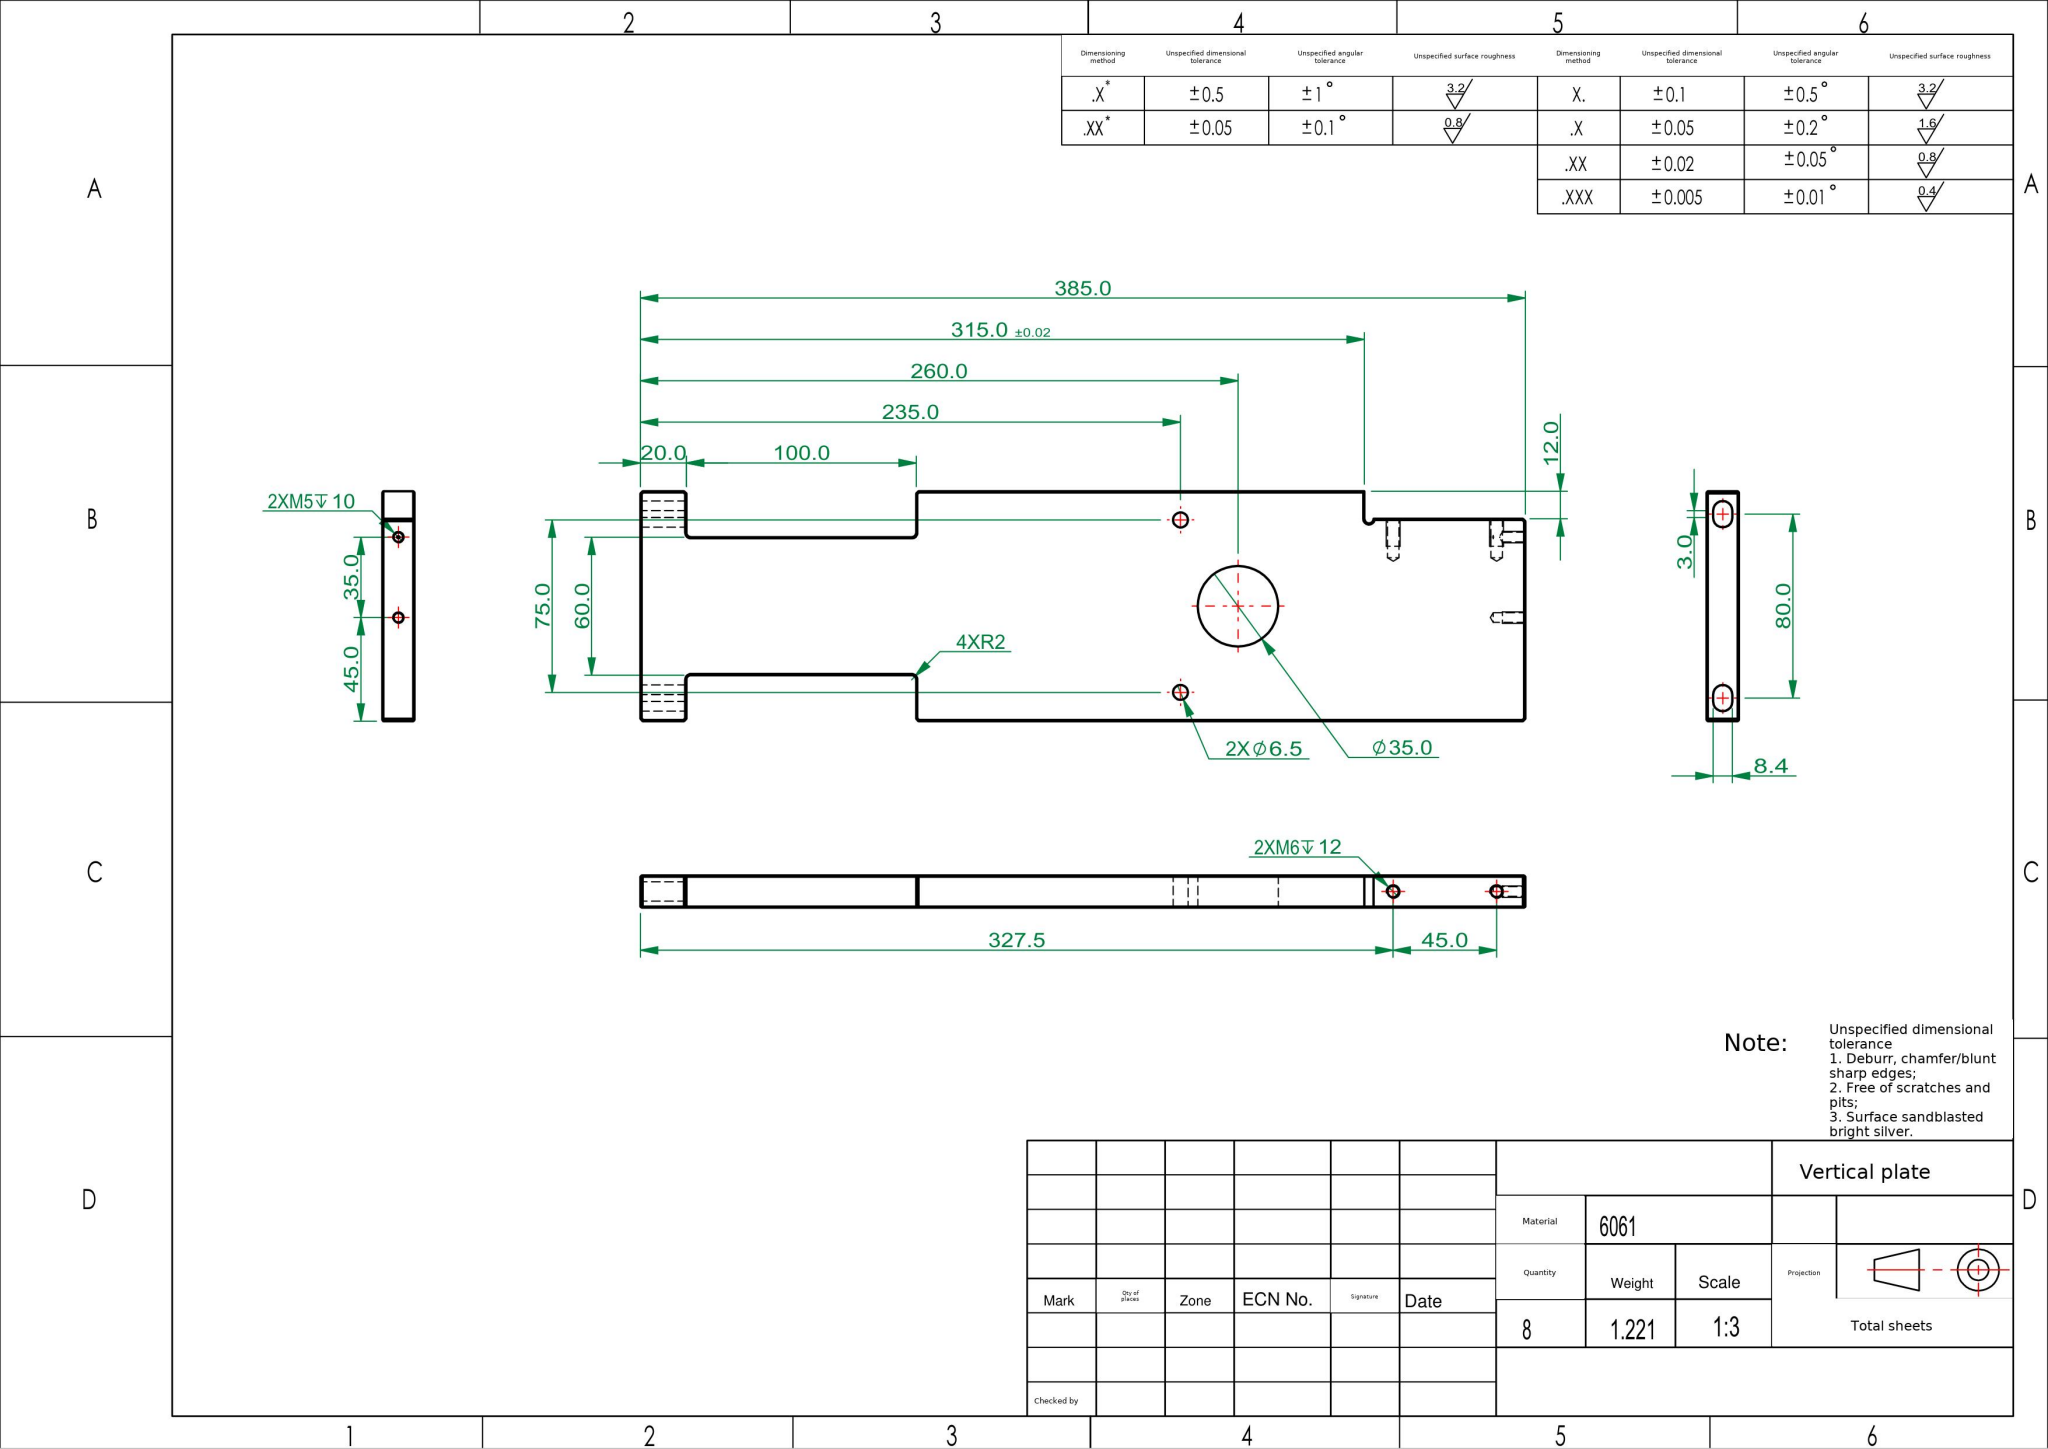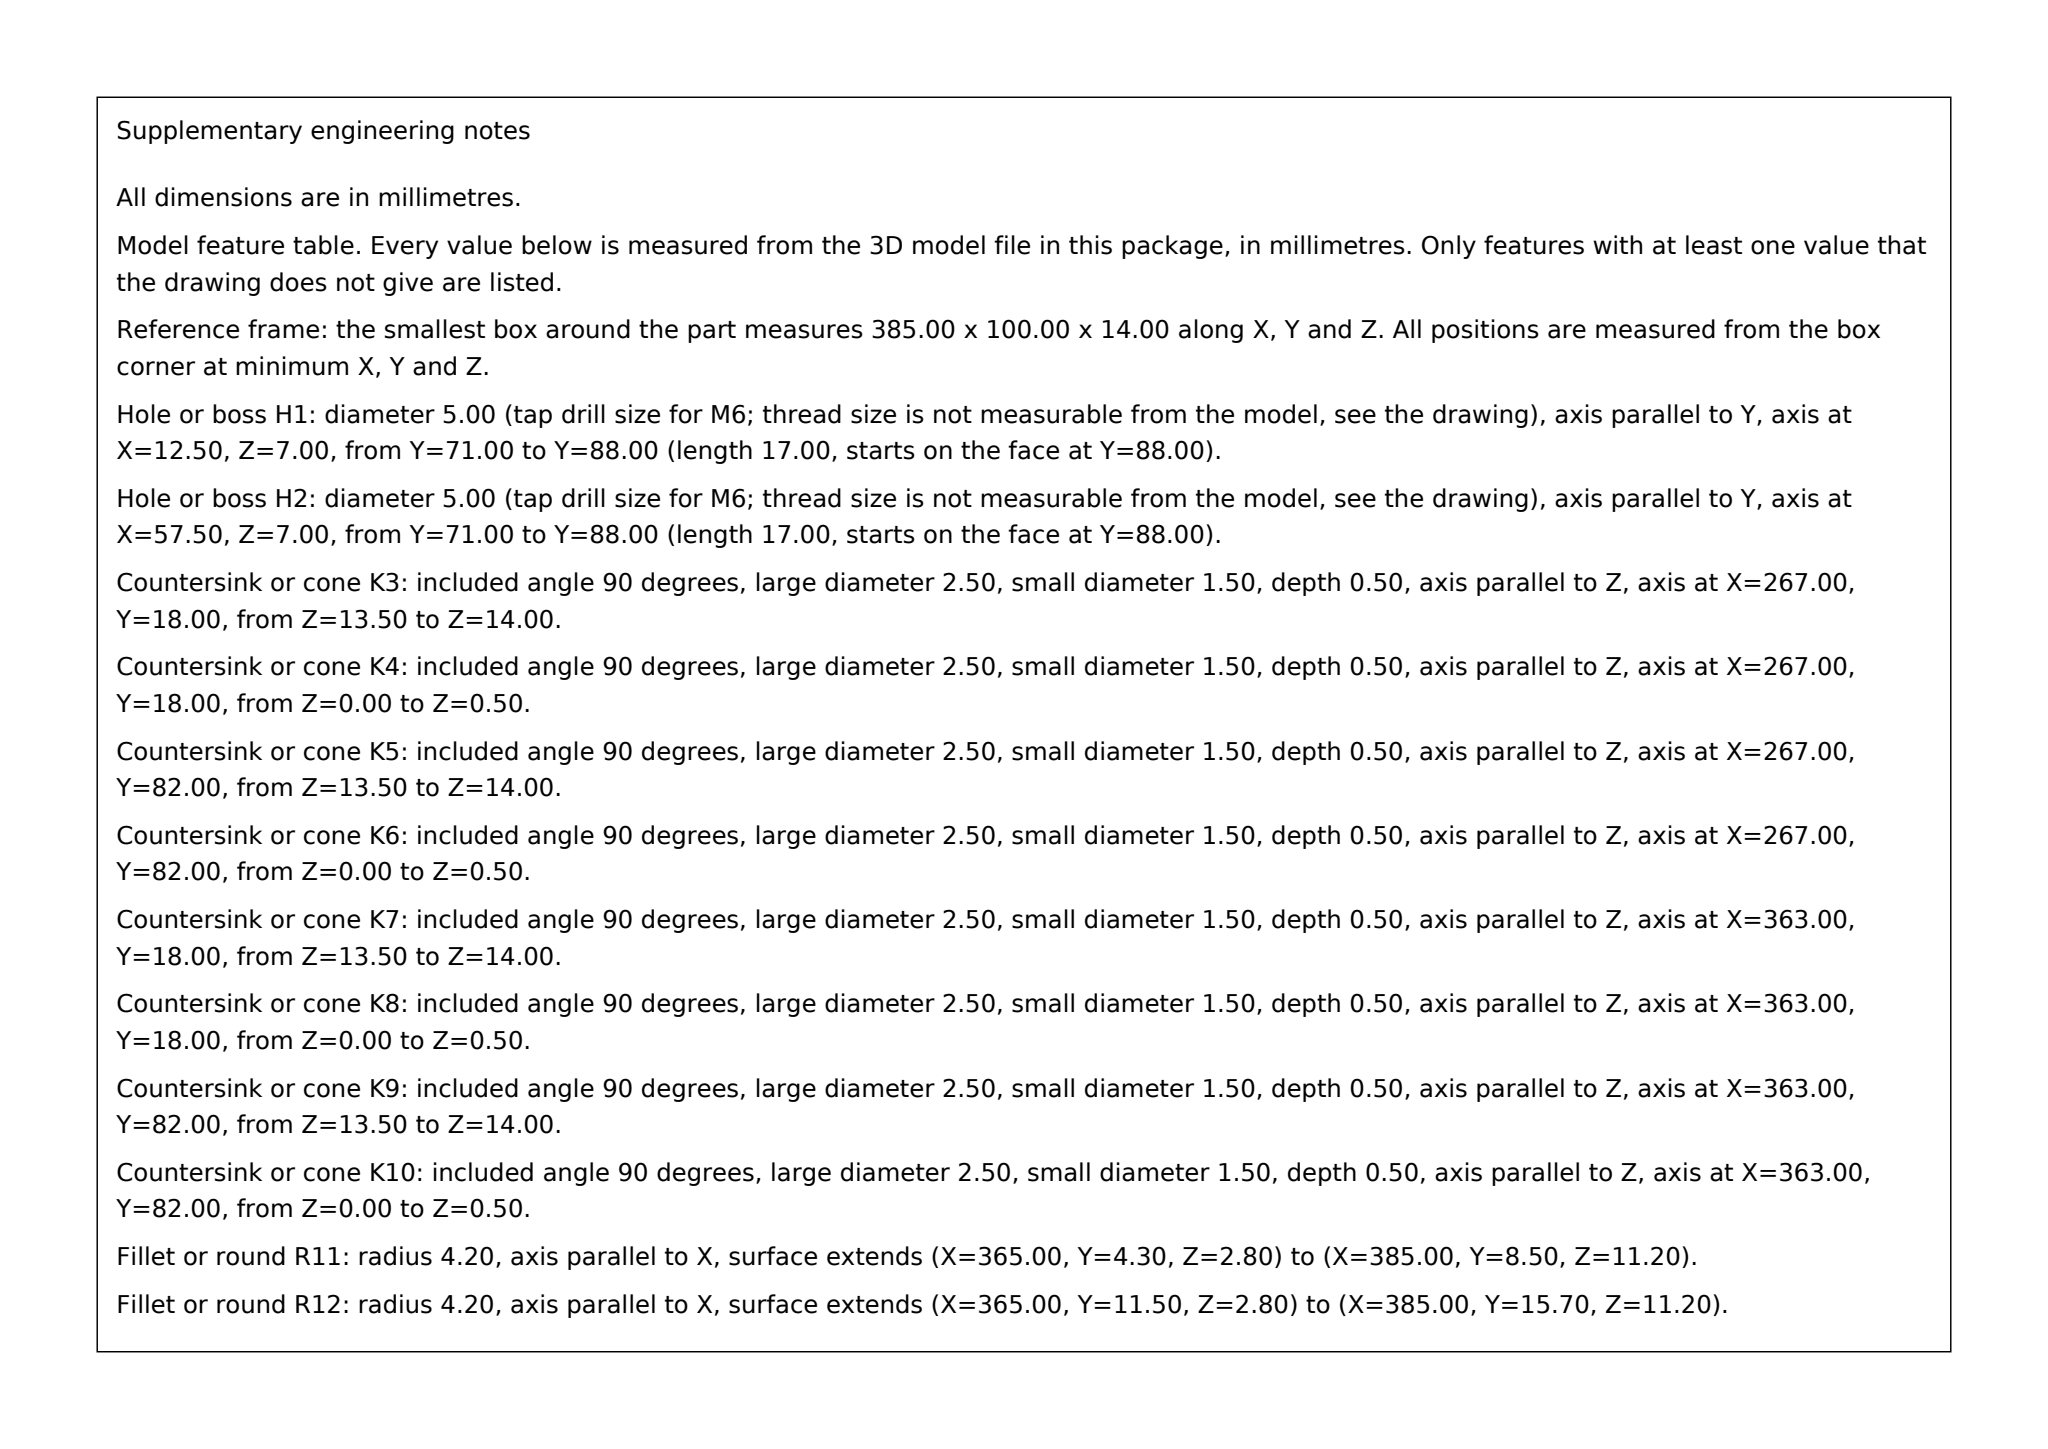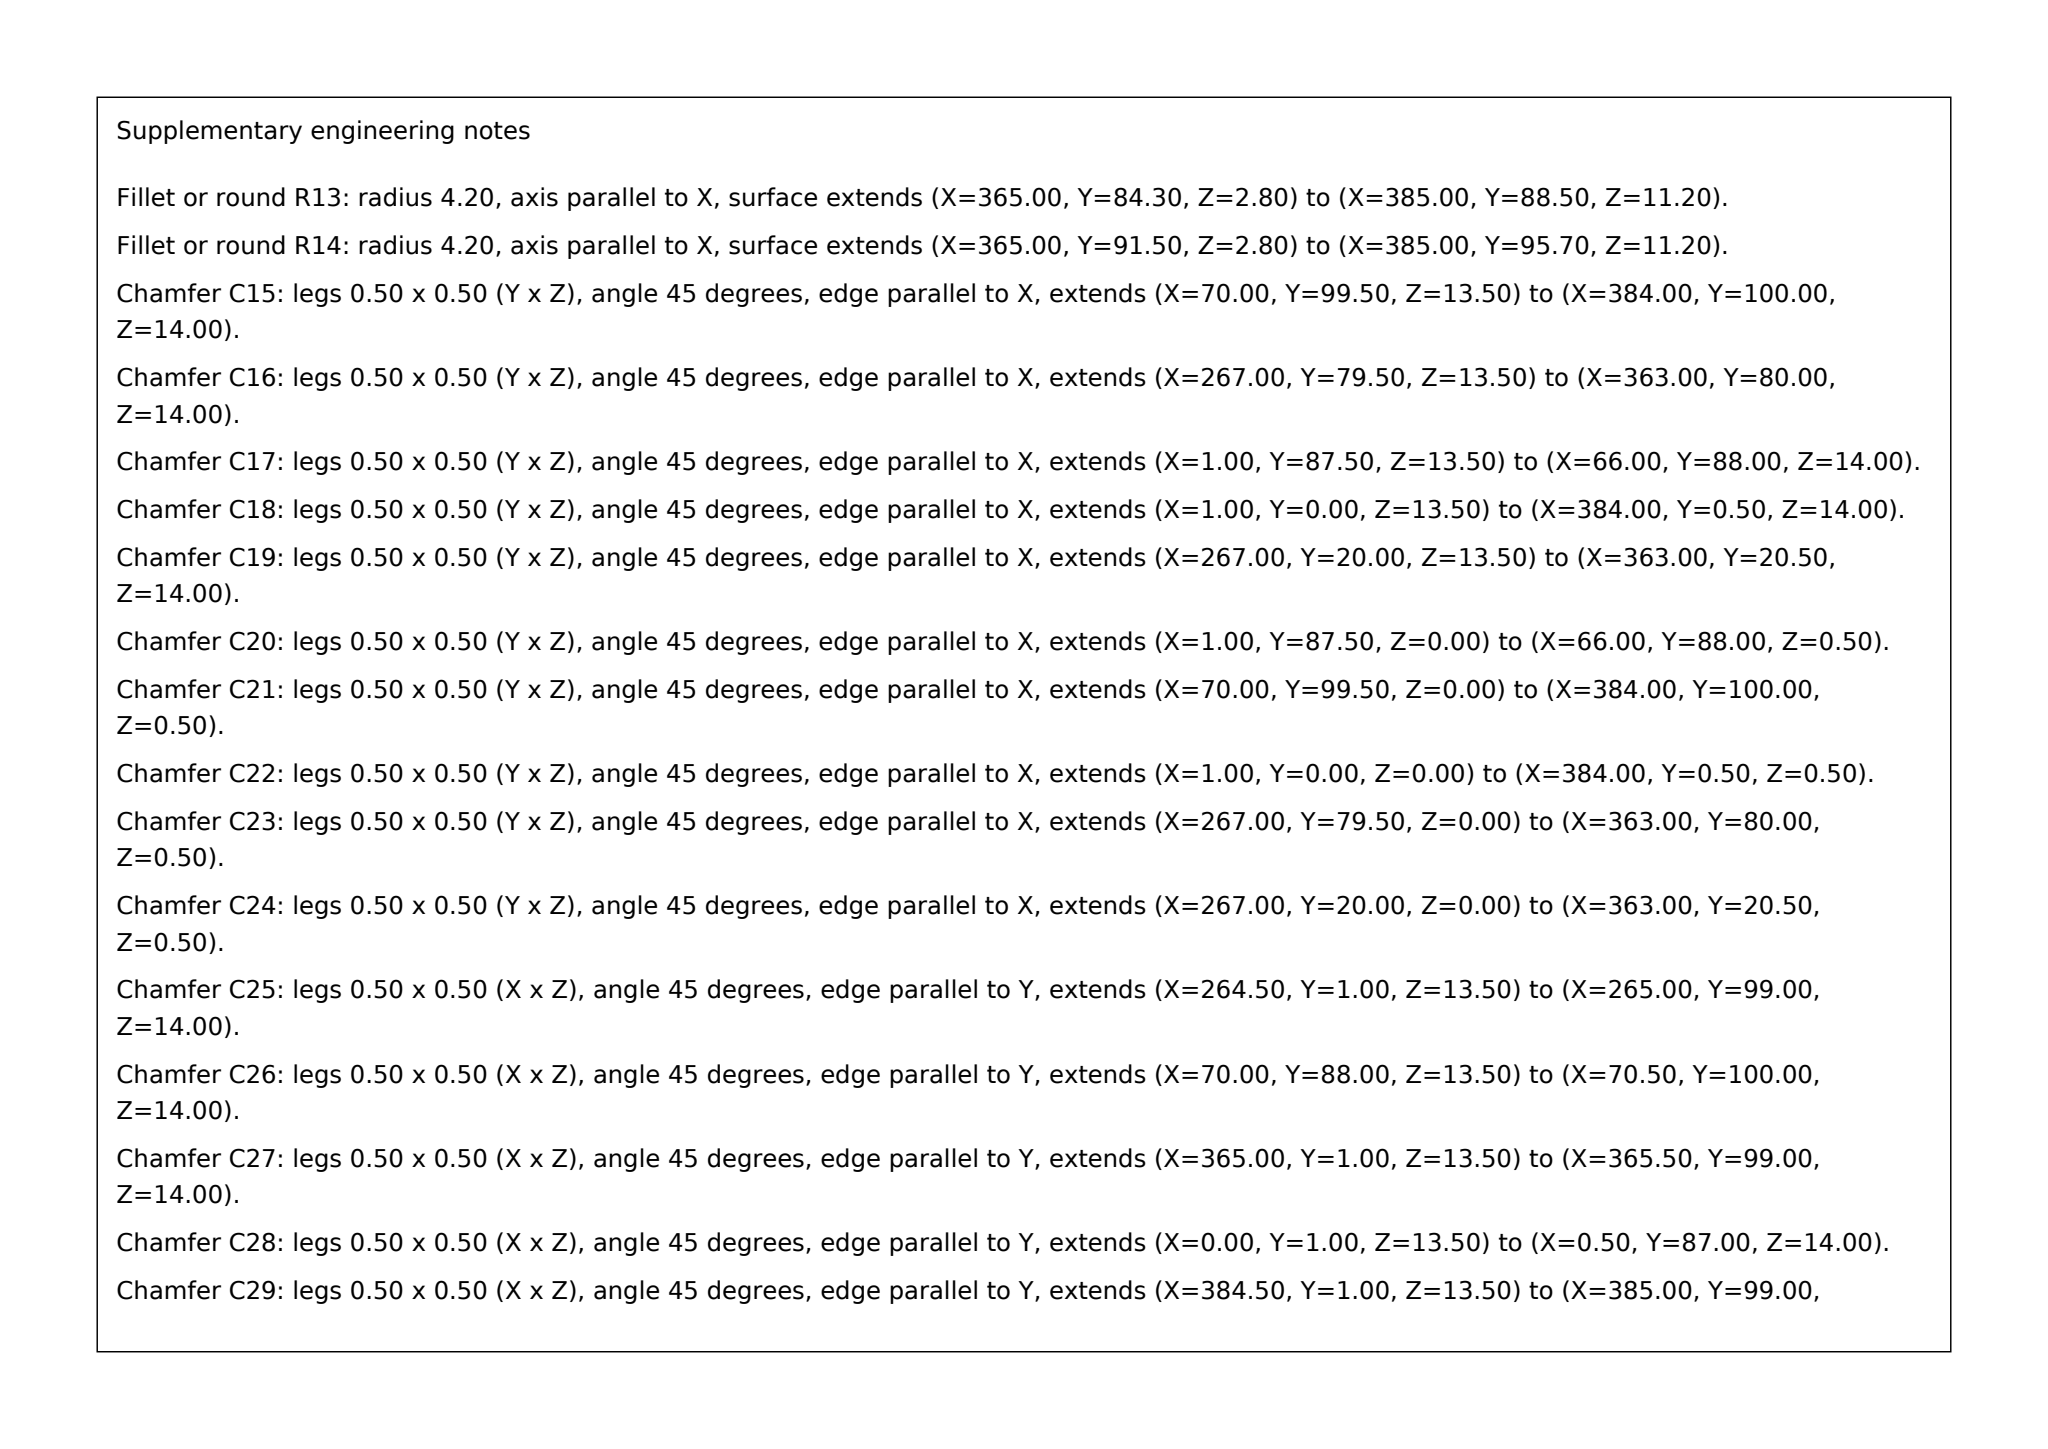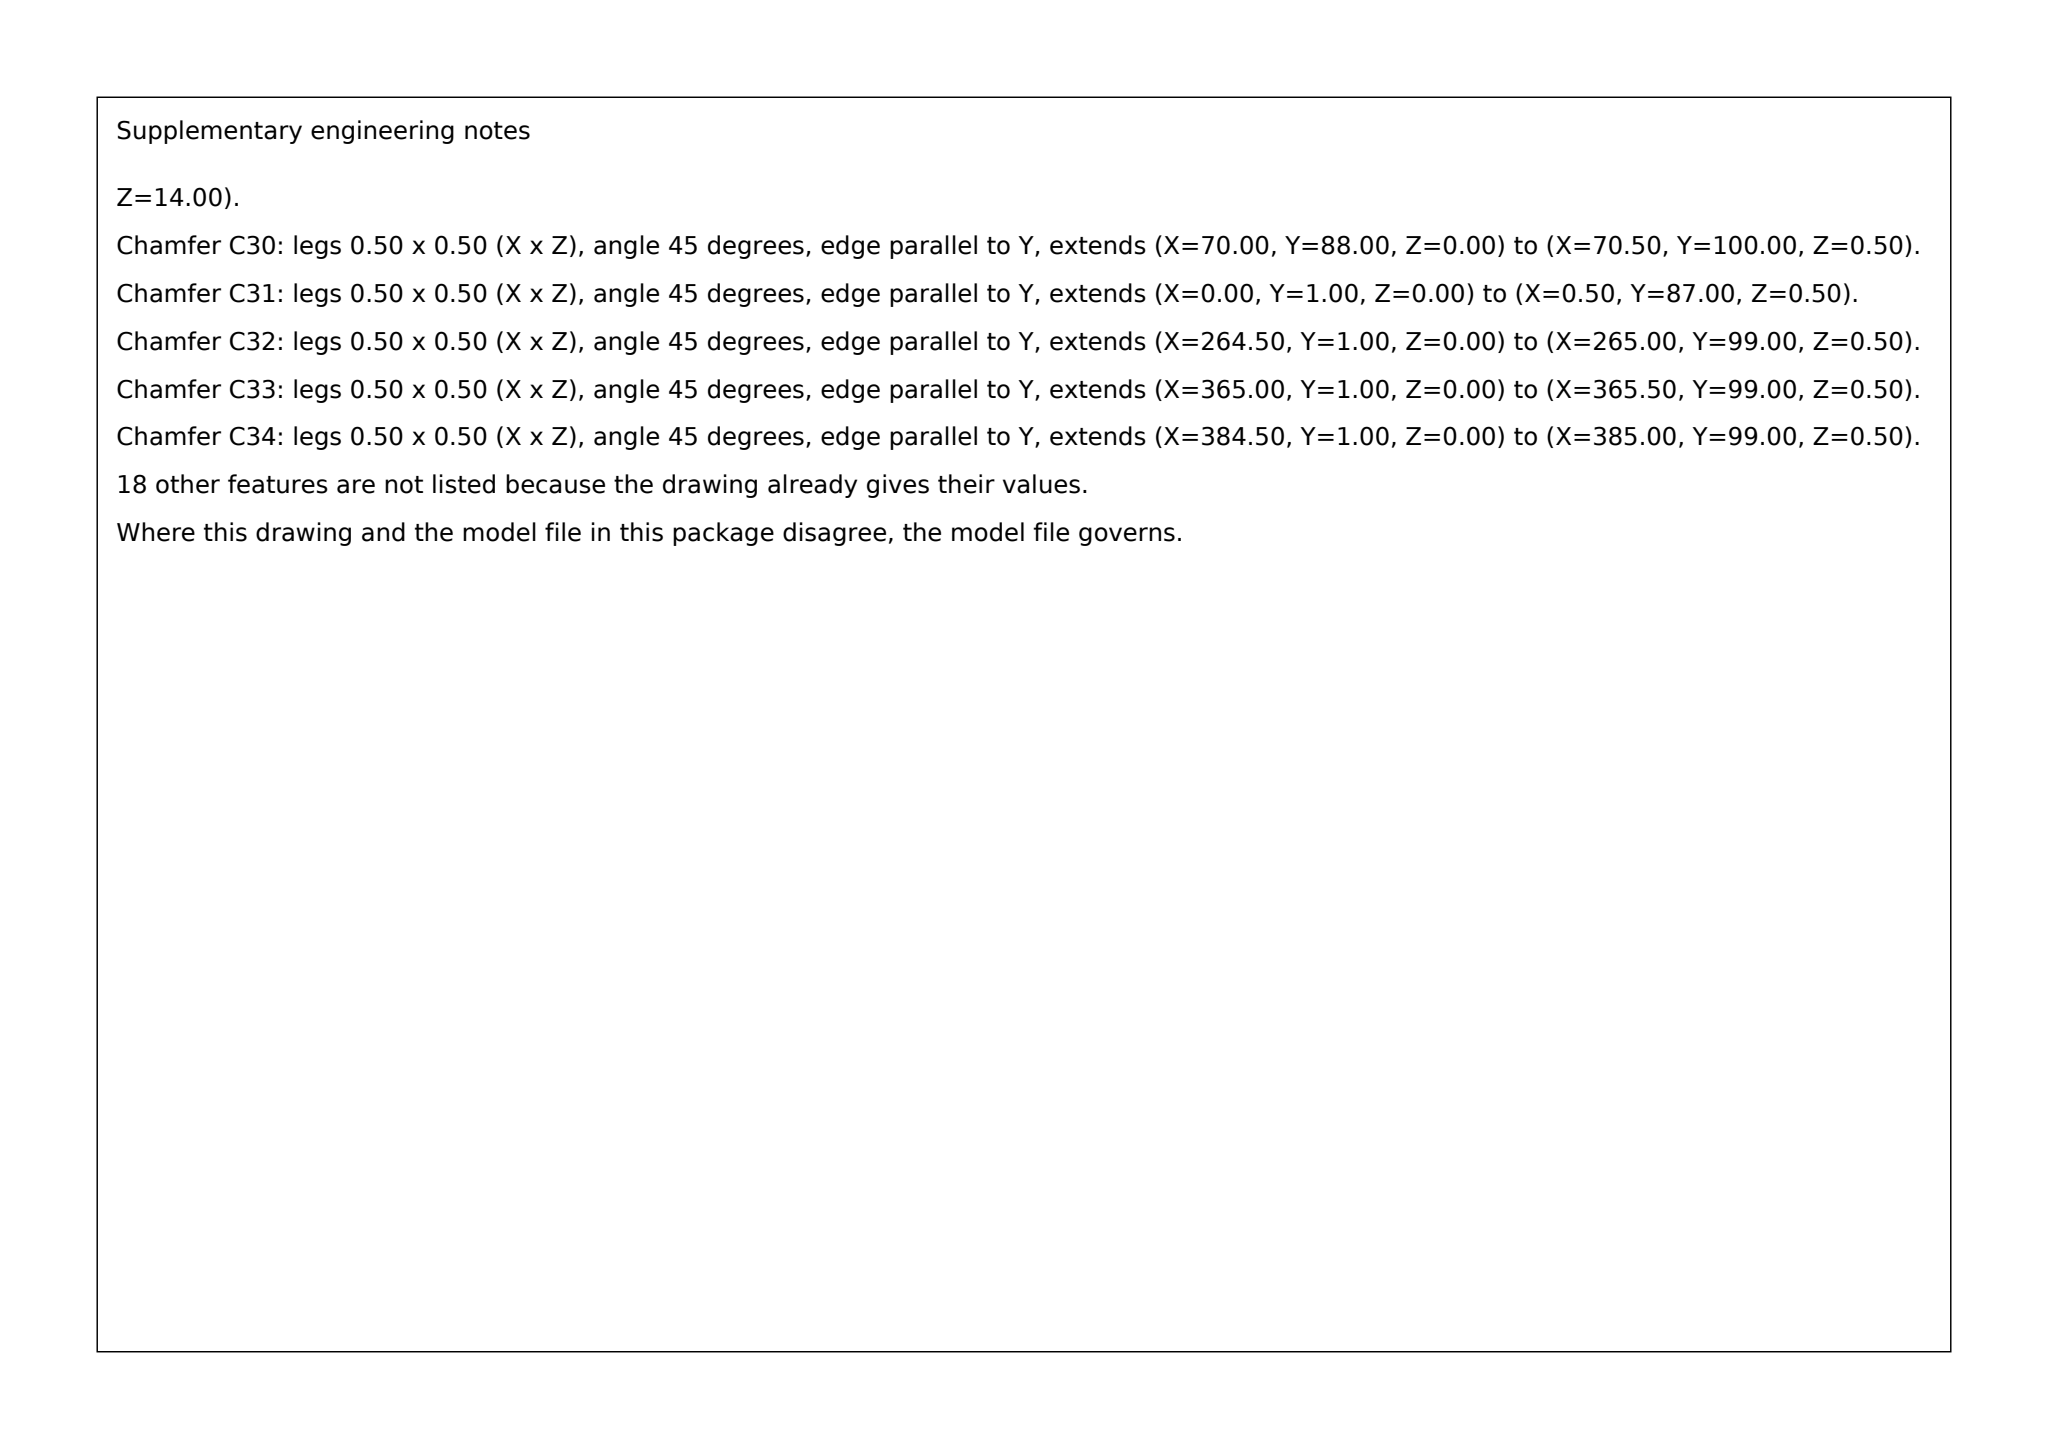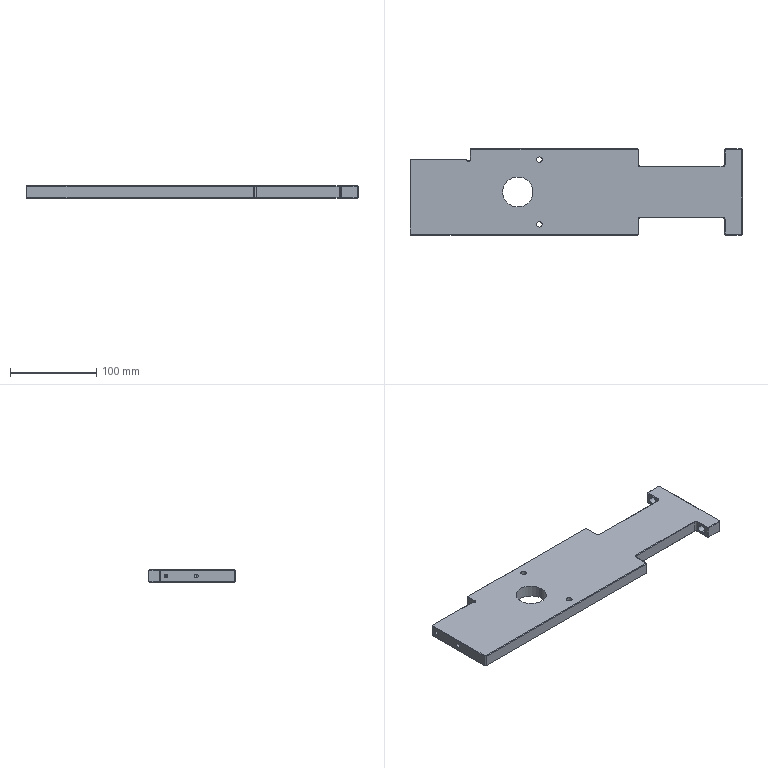Part | SolidWorks | mm | material 6061 | 1 solid | 121 faces | box 385 x 100 x 14 mm | volume 452231 mm3 | plane 72 | cylinder 28 | cone 21 | commonest cylinder face diameters 4.2 x7 8.4 x6 4 x5 6.5 x4 5 x4 35 x2
build123d program:
from build123d import *

# Parameters (mm, degrees)
SKETCH1_W                      = 385
SKETCH1_H                      = 100
BOSS_EXTRUDE1_DEPTH            = 7
SKETCH2_W                      = 100
SKETCH2_H                      = 20
CUT_EXTRUDE1_DEPTH             = 70
SKETCH3_W                      = 70
SKETCH3_H                      = 12
CUT_EXTRUDE2_DEPTH             = 70
M6_TAPPED_HOLE1_D              = 5
M6_TAPPED_HOLE1_DEPTH          = 17
M6_TAPPED_HOLE1_TIP            = 1.502
F_8_4_8_4_DIAMETER_HOLE1_D     = 8.4
F_8_4_8_4_DIAMETER_HOLE1_DEPTH = 20
SKETCH8_R                      = 2
CUT_EXTRUDE3_DEPTH             = 31
FILLET1_R                      = 2
CHAMFER1_SIZE                  = 1
CHAMFER2_SIZE                  = 0.5
CUT_EXTRUDE4_DEPTH             = 25
F_6_5_6_5_DIAMETER_HOLE1_D     = 6.5
F_6_5_6_5_DIAMETER_HOLE1_DEPTH = 20
F_6_5_6_5_DIAMETER_HOLE1_TIP   = 1.953
M5_TAPPED_HOLE1_D              = 4.2
M5_TAPPED_HOLE1_DEPTH          = 14
M5_TAPPED_HOLE1_TIP            = 1.262
SKETCH14_R                     = 17.5
CUT_EXTRUDE5_DEPTH             = 116


with BuildPart() as part:
    # Sketch1 → Boss-Extrude1 (new, symmetric)
    with BuildSketch(Plane.XY):
        Rectangle(SKETCH1_W, SKETCH1_H)
    extrude(amount=BOSS_EXTRUDE1_DEPTH, both=True)

    # Sketch2 → Cut-Extrude1 (cut)
    with BuildSketch(Plane.XY.offset(7)):
        with Locations((122.5, 40)):
            Rectangle(SKETCH2_W, SKETCH2_H)
        with Locations((122.5, -40)):
            Rectangle(SKETCH2_W, SKETCH2_H)
    extrude(amount=-CUT_EXTRUDE1_DEPTH, mode=Mode.SUBTRACT)

    # Sketch3 → Cut-Extrude2 (cut)
    with BuildSketch(Plane.XY.offset(7)):
        with Locations((-157.5, 44)):
            Rectangle(SKETCH3_W, SKETCH3_H)
    extrude(amount=-CUT_EXTRUDE2_DEPTH, mode=Mode.SUBTRACT)

    # M6 Tapped Hole1
    with Locations(Plane(origin=(-180, 38, 0), x_dir=(0, 0, 1), z_dir=(0, 1, 0))):
        with Locations((0, 0), (0, 45)):
            Hole(M6_TAPPED_HOLE1_D / 2, depth=M6_TAPPED_HOLE1_DEPTH)
            with Locations((0, 0, -(M6_TAPPED_HOLE1_DEPTH + M6_TAPPED_HOLE1_TIP / 2))):  # 118° drill point
                Cone(0, M6_TAPPED_HOLE1_D / 2, M6_TAPPED_HOLE1_TIP, mode=Mode.SUBTRACT)

    # 8.4 _8.4_ Diameter Hole1
    with Locations(Plane(origin=(172.5, 40, 0), x_dir=(0, -1, 0), z_dir=(-1, 0, 0))):
        with Locations((0, 0), (80, 0)):
            Hole(F_8_4_8_4_DIAMETER_HOLE1_D / 2, depth=F_8_4_8_4_DIAMETER_HOLE1_DEPTH)

    # Sketch8 → Cut-Extrude3 (cut)
    with BuildSketch(Plane(origin=(0, 0, -7), x_dir=(-1, 0, 0), z_dir=(0, 0, -1))):
        with Locations((124.5, 38)):
            Circle(SKETCH8_R)
    extrude(amount=-CUT_EXTRUDE3_DEPTH, mode=Mode.SUBTRACT)

    # Fillet1
    fillet1_edges = [part.edges().sort_by_distance(p)[0] for p in [
        (172.5, 30, 0),
        (72.5, 30, 0),
        (172.5, -30, 0),
        (72.5, -30, 0),
    ]]
    fillet(fillet1_edges, radius=FILLET1_R)

    # Chamfer1
    chamfer1_edges = [part.edges().sort_by_distance(p)[0] for p in [
        (172.5, 50, 0),
        (72.5, 50, 0),
        (172.5, -50, 0),
        (72.5, -50, 0),
        (-192.5, 38, 0),
        (192.5, -50, 0),
        (-192.5, -50, 0),
        (192.5, 50, 0),
    ]]
    chamfer(chamfer1_edges, length=CHAMFER1_SIZE)

    # Chamfer2
    chamfer2_edges = [part.edges().sort_by_distance(p)[0] for p in [
        (72.5, -40.5, 7),
        (72.5, -40.5, -7),
        (122.5, 30, 7),
        (122.5, 30, -7),
        (172.5, 40.5, 7),
        (172.5, 40.5, -7),
        (171.914, -30.586, 7),
        (171.914, -30.586, -7),
        (73.086, -30.586, 7),
        (73.086, -30.586, -7),
        (73.086, 30.586, 7),
        (73.086, 30.586, -7),
        (171.914, 30.586, 7),
        (171.914, 30.586, -7),
        (172.5, -40.5, 7),
        (172.5, -40.5, -7),
        (-159, 38, 7),
        (-192.5, -6, 7),
        (-60, -50, 7),
        (182.5, -50, 7),
        (192.5, 0, 7),
        (182.5, 50, 7),
        (72.5, 40.5, 7),
        (-25.5, 50, 7),
        (-192, -49.5, 7),
        (72, -49.5, 7),
        (72, 49.5, 7),
        (-192, 37.5, 7),
        (192, -49.5, 7),
        (192, 49.5, 7),
        (173, 49.5, 7),
        (173, -49.5, 7),
        (182.5, -50, -7),
        (-159, 38, -7),
        (-25.5, 50, -7),
        (72.5, 40.5, -7),
        (182.5, 50, -7),
        (192.5, 0, -7),
        (-60, -50, -7),
        (-192.5, -6, -7),
        (-192, -49.5, -7),
        (72, -49.5, -7),
        (72, 49.5, -7),
        (-192, 37.5, -7),
        (192, -49.5, -7),
        (192, 49.5, -7),
        (173, 49.5, -7),
        (173, -49.5, -7),
        (-122.5, 44, -7),
        (-122.5, 44, 7),
        (-124.5, 36, -7),
        (-124.5, 36, 7),
        (122.5, -30, 7),
        (122.5, -30, -7),
    ]]
    chamfer(chamfer2_edges, length=CHAMFER2_SIZE)

    # Sketch9 → Cut-Extrude4 (cut)
    with BuildSketch(Plane(origin=(192.5, 0, 0), x_dir=(0, 0, -1), z_dir=(1, 0, 0))):
        with BuildLine():
            Line((-4.2, 38.5), (-4.2, 41.5))
            ThreePointArc((-4.2, 41.5), (0, 45.7), (4.2, 41.5))
            Line((4.2, 41.5), (4.2, 38.5))
            ThreePointArc((4.2, 38.5), (0, 34.3), (-4.2, 38.5))
        make_face()
        with BuildLine():
            Line((-4.2, -41.5), (-4.2, -38.5))
            ThreePointArc((-4.2, -38.5), (0, -34.3), (4.2, -38.5))
            Line((4.2, -38.5), (4.2, -41.5))
            ThreePointArc((4.2, -41.5), (0, -45.7), (-4.2, -41.5))
        make_face()
    extrude(amount=-CUT_EXTRUDE4_DEPTH, mode=Mode.SUBTRACT)

    # 6.5 _6.5_ Diameter Hole1
    with Locations(Plane(origin=(-42.5, 37.5, -7), x_dir=(-1, 0, 0), z_dir=(0, 0, -1))):
        with Locations((0, 0), (0, -75)):
            Hole(F_6_5_6_5_DIAMETER_HOLE1_D / 2, depth=F_6_5_6_5_DIAMETER_HOLE1_DEPTH)
            with Locations((0, 0, -(F_6_5_6_5_DIAMETER_HOLE1_DEPTH + F_6_5_6_5_DIAMETER_HOLE1_TIP / 2))):  # 118° drill point
                Cone(0, F_6_5_6_5_DIAMETER_HOLE1_D / 2, F_6_5_6_5_DIAMETER_HOLE1_TIP, mode=Mode.SUBTRACT)

    # M5 Tapped Hole1
    with Locations(Plane(origin=(-192.5, 30, 0), x_dir=(0, -1, 0), z_dir=(-1, 0, 0))):
        with Locations((0, 0), (35, 0)):
            Hole(M5_TAPPED_HOLE1_D / 2, depth=M5_TAPPED_HOLE1_DEPTH)
            with Locations((0, 0, -(M5_TAPPED_HOLE1_DEPTH + M5_TAPPED_HOLE1_TIP / 2))):  # 118° drill point
                Cone(0, M5_TAPPED_HOLE1_D / 2, M5_TAPPED_HOLE1_TIP, mode=Mode.SUBTRACT)

    # Sketch14 → Cut-Extrude5 (cut)
    with BuildSketch(Plane(origin=(0, 0, -7), x_dir=(-1, 0, 0), z_dir=(0, 0, -1))):
        with Locations((67.5, 0)):
            Circle(SKETCH14_R)
    extrude(amount=-CUT_EXTRUDE5_DEPTH, mode=Mode.SUBTRACT)


solid = part.part